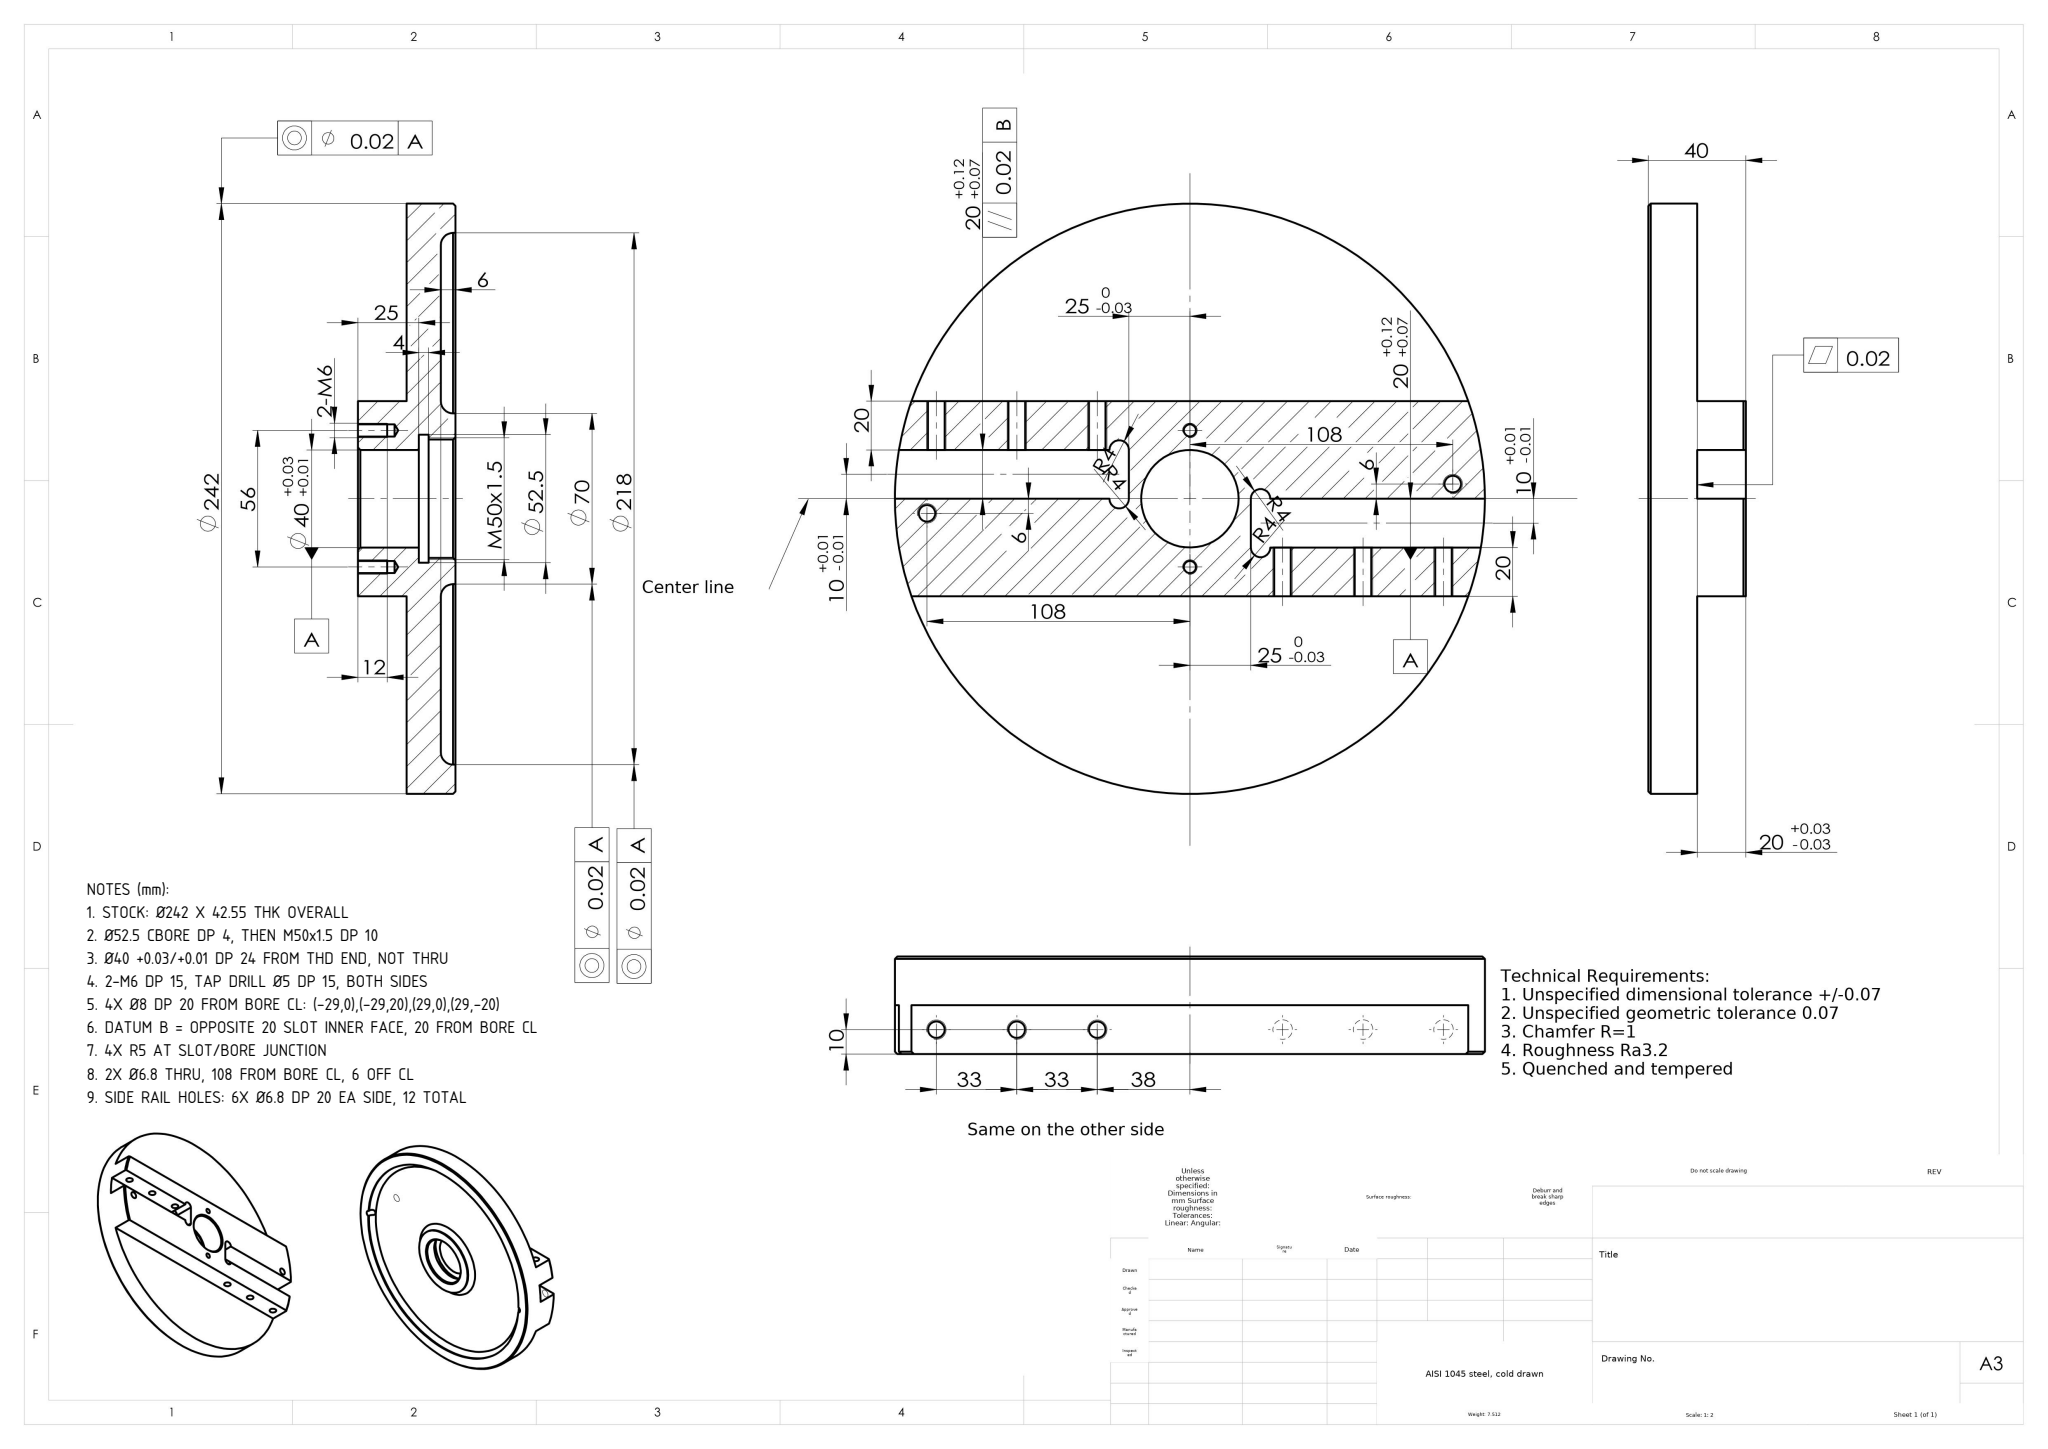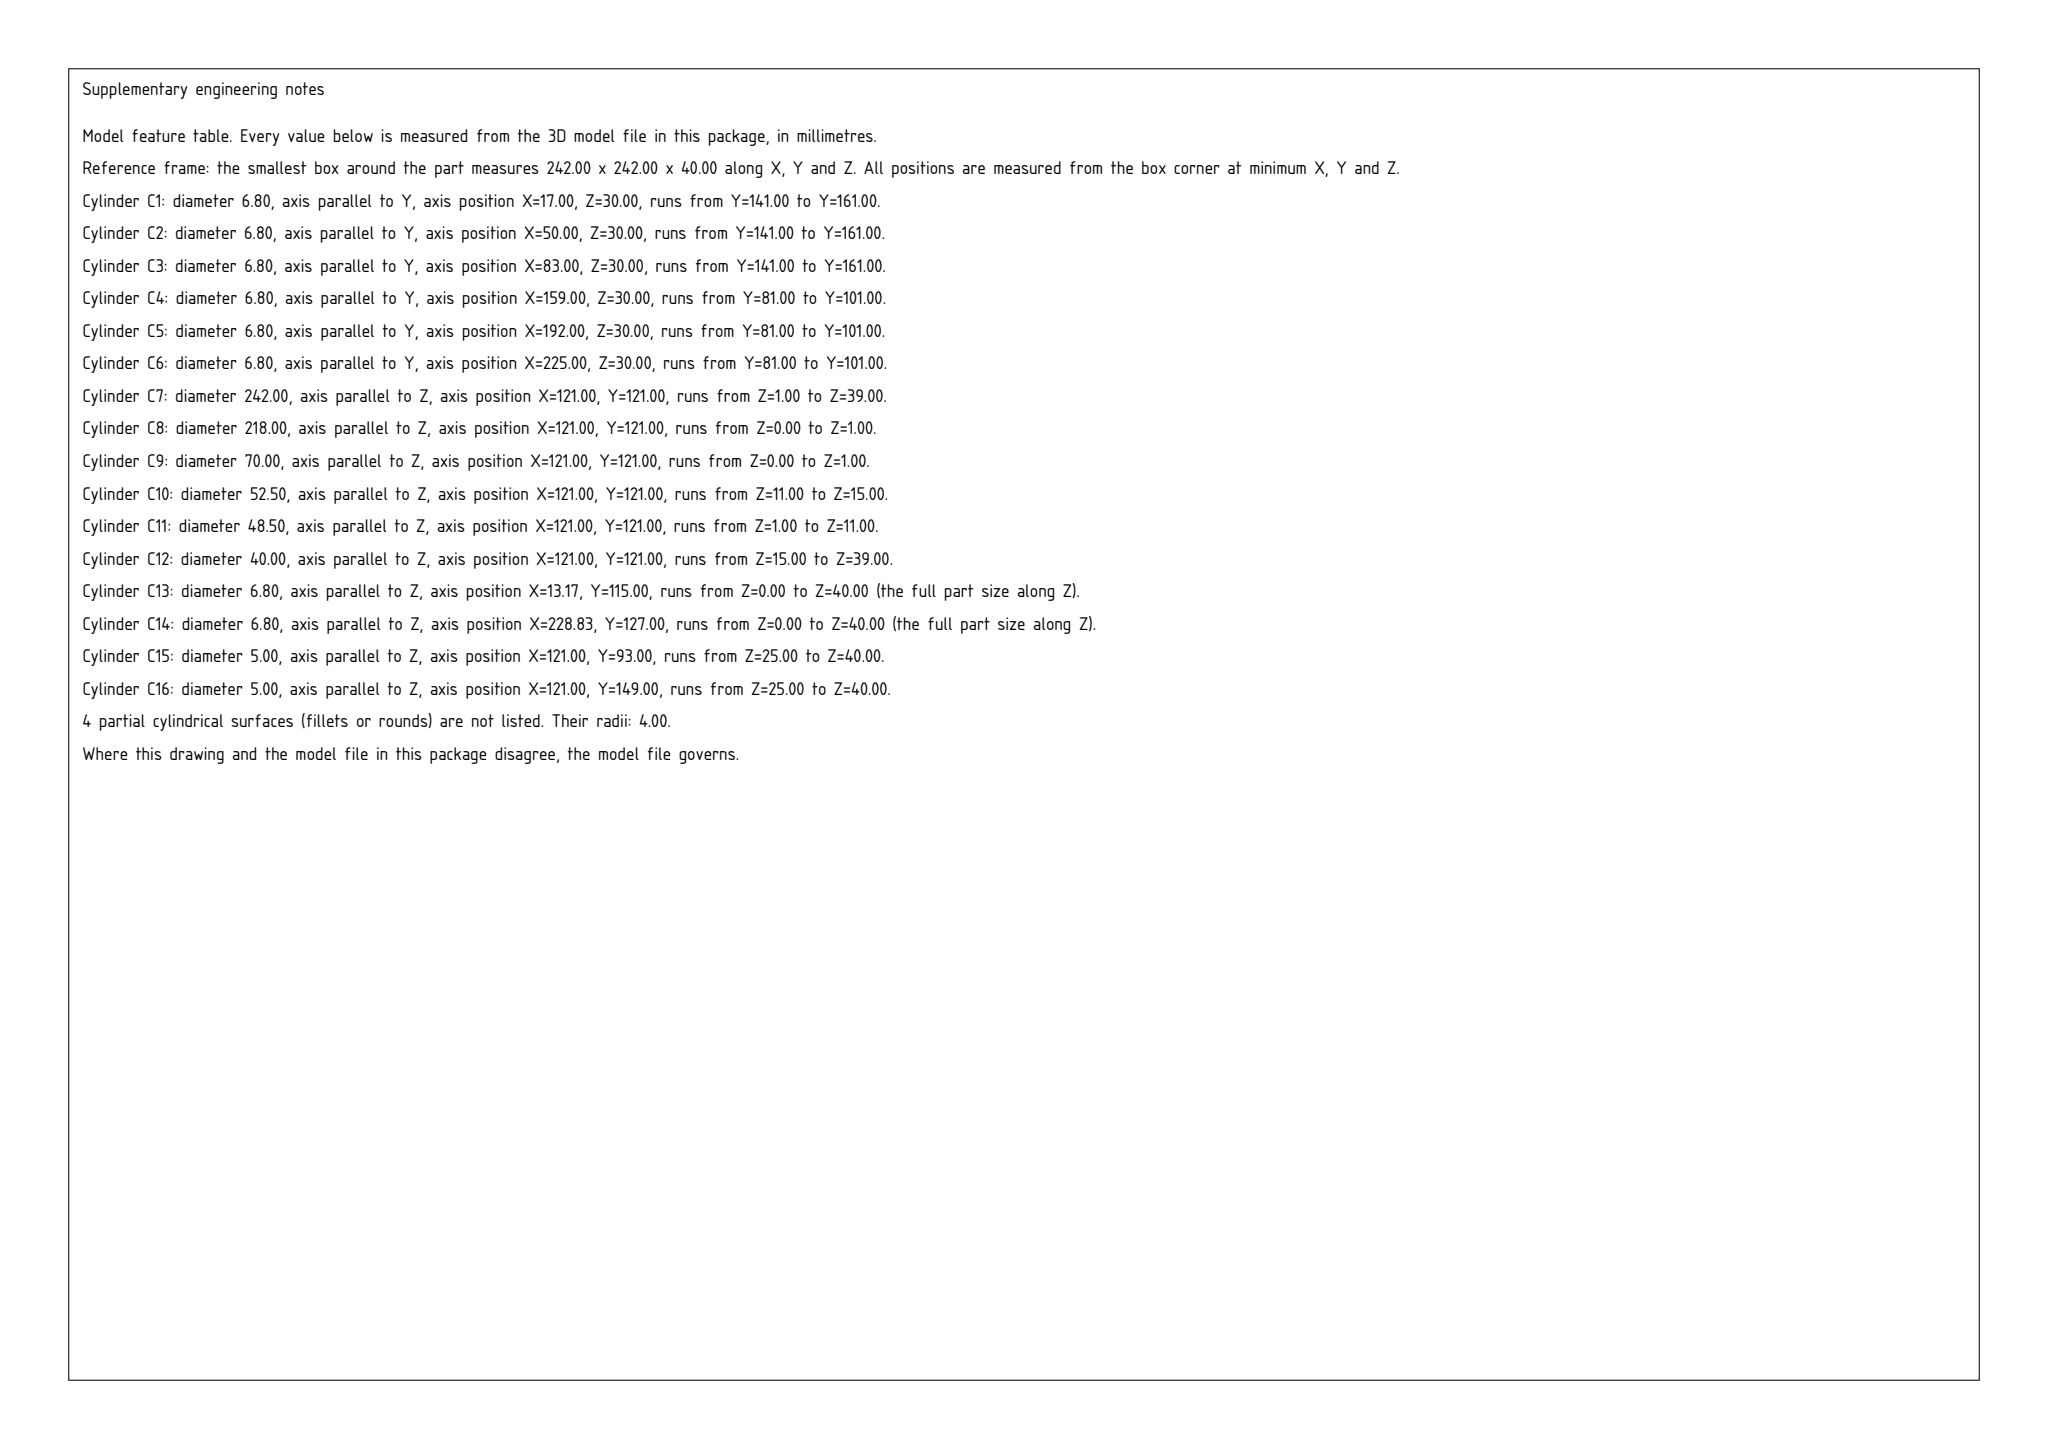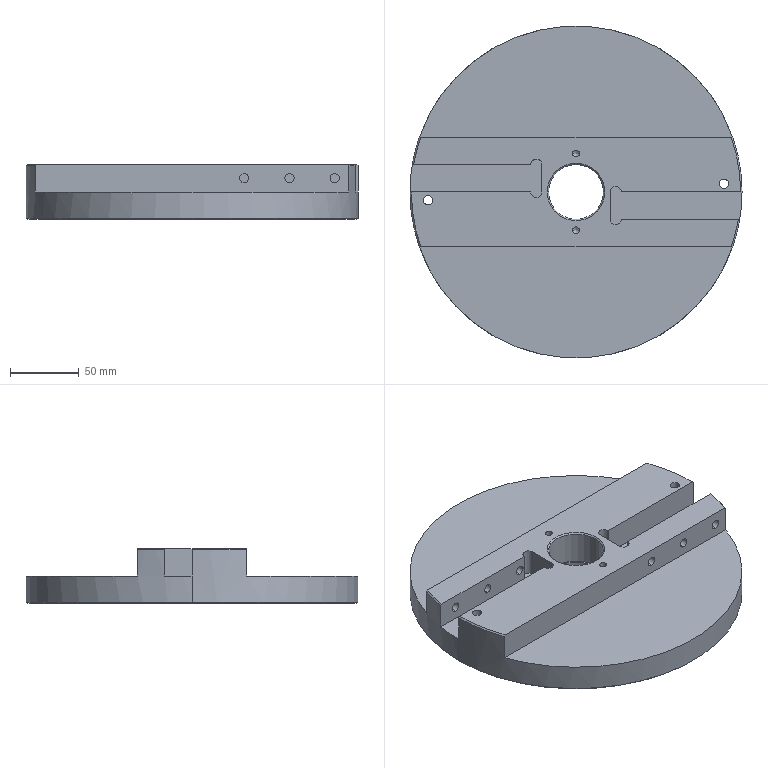Part | SolidWorks | mm | 1 solid | 73 faces | box 242 x 242 x 40 mm | volume 956950 mm3 | cylinder 37 | plane 18 | cone 14 | torus 4 | commonest cylinder face diameters 6.8 x16 5 x4 8 x4 218 x3 70 x2 52.5 x2 48.5 x2 40 x2
Drawing notes:
STOCK: Ø242 X 42.55 THK OVERALL | from the solid: bbox_xyz 242.0 x 242.0 x 42.55; Ø242 z-cyl L=38 at (121,121)
Ø52.5 CBORE DP 4, THEN M50x1.5 DP 10 | from the solid: dia 52.5 z-cyl L=4 then dia 48.5 (thd minor) z-cyl L=10, both at (121,121)
Ø40 +0.03/+0.01 DP 24 FROM THD END, NOT THRU | from the solid: dia 40.0 z-cyl at (121,121) L=24; 24 < 42.55 bbox z; 90° cone ref dia 40
2-M6 DP 15, TAP DRILL Ø5 DP 15, BOTH SIDES | from the solid: Ø5 z-cyls at (121,93) & (121,149) L=15, count 2 each; 118° drill cones ref dia 5
4X Ø8 DP 20 FROM BORE CL: (-29,0),(-29,20),(29,0),(29,-20) | from the solid: Ø8 z-cyls L=20 at (92,121),(92,141),(150,101),(150,121); bore CL (121,121)
DATUM B = OPPOSITE 20 SLOT INNER FACE, 20 FROM BORE CL | from the solid: y-planes at 101 and 141 = ±20 from bore CL y=121; slots y 81-101 and 141-161
4X R5 AT SLOT/BORE JUNCTION | from the solid: fillet_radii [5.0, qty 4]
2X Ø6.8 THRU, 108 FROM BORE CL, 6 OFF CL | from the solid: Ø6.8 z-cyls L=40 (thru) at (13.17,115) & (228.83,127); bore CL (121,121)
SIDE RAIL HOLES: 6X Ø6.8 DP 20 EA SIDE, 12 TOTAL | from the solid: Ø6.8 y-cyls L=20 at x=17,50,83,159,192,225, z=32.55, count 2 each